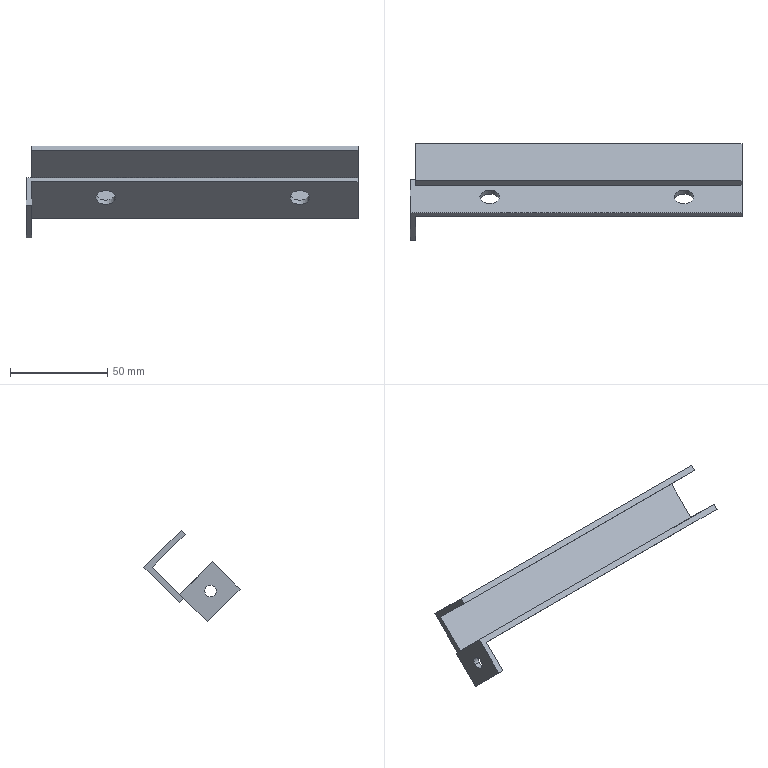Component | SolidWorks | LeftGuardBracket-1 | 1 solid | 20 faces | box 171 x 49.5 x 47.34 mm | volume 38177 mm3 | plane 14 | cylinder 6 | commonest cylinder face diameters 10 x4 6 x2
build123d program:
from build123d import *

# Parameters (mm, degrees)
EXTRUDE_THIN1_DEPTH = 168
SKETCH2_W           = 23.953
SKETCH2_H           = 20
BOSS_EXTRUDE1_DEPTH = 3
SKETCH3_R           = 5
CUT_EXTRUDE1_DEPTH  = 3
SKETCH4_R           = 3
CUT_EXTRUDE2_DEPTH  = 3


with BuildPart() as part:
    # Sketch1 → Extrude-Thin1 (new body)
    with BuildSketch(Plane.XY):
        Polygon((3.367, -34.031), (-23.633, -34.031), (-23.633, -8.031), (3.367, -8.031), (3.367, -11.031), (-20.633, -11.031), (-20.633, -31.031), (3.367, -31.031), align=None)
    extrude(amount=EXTRUDE_THIN1_DEPTH)

    # Sketch2 → Boss-Extrude1 (add)
    with BuildSketch(Plane.XY.offset(168)):
        with Locations((-8.609, -41.031)):
            Rectangle(SKETCH2_W, SKETCH2_H)
    extrude(amount=BOSS_EXTRUDE1_DEPTH)

    # Sketch3 → Cut-Extrude1 (cut)
    with BuildSketch(Plane(origin=(0, -34.031, 0), x_dir=(-1, 0, 0), z_dir=(0, -1, 0))):
        with Locations(Location((8.109, -130, 0), (0, 0, 90))):
            Circle(SKETCH3_R)
        with Locations(Location((8.109, -30, 0), (0, 0, 90))):
            Circle(SKETCH3_R)
    extrude(amount=-CUT_EXTRUDE1_DEPTH, mode=Mode.SUBTRACT)

    # Sketch4 → Cut-Extrude2 (cut)
    with BuildSketch(Plane.XY.offset(171)):
        with Locations((-8.109, -41.031)):
            Circle(SKETCH4_R)
    extrude(amount=-CUT_EXTRUDE2_DEPTH, mode=Mode.SUBTRACT)


solid = part.part

# Placed as in the assembly
solid = solid.moved(Location((-271.55, -172.786, -218.111), (45, -90, 0)))
STEP:
#1=COLOUR_RGB('',0.7922,0.8196,0.9333);
#2=FILL_AREA_STYLE_COLOUR('',#1);
#3=FILL_AREA_STYLE('',(#2));
#4=SURFACE_STYLE_FILL_AREA(#3);
#5=SURFACE_SIDE_STYLE('',(#4));
#6=SURFACE_STYLE_USAGE(.BOTH.,#5);
#7=PRESENTATION_STYLE_ASSIGNMENT((#6));
#8=CARTESIAN_POINT('',(-17.305,-7.636,-10.039));
#9=VERTEX_POINT('',#8);
#10=CARTESIAN_POINT('',(-17.305,-7.803,-9.872));
#11=VERTEX_POINT('',#10);
#12=CARTESIAN_POINT('',(-17.305,-7.719,-9.955));
#13=DIRECTION('',(-1.,0.,0.));
#14=DIRECTION('',(0.,-0.7071,0.7071));
#15=AXIS2_PLACEMENT_3D('',#12,#13,#14);
#16=CIRCLE('',#15,0.1181);
#17=EDGE_CURVE('',#9,#11,#16,.T.);
#18=ORIENTED_EDGE('',*,*,#17,.F.);
#19=CARTESIAN_POINT('',(-17.423,-7.636,-10.039));
#20=VERTEX_POINT('',#19);
#21=CARTESIAN_POINT('',(-17.305,-7.636,-10.039));
#22=DIRECTION('',(-1.,0.,0.));
#23=VECTOR('',#22,39.37);
#24=LINE('',#21,#23);
#25=EDGE_CURVE('',#9,#20,#24,.T.);
#26=ORIENTED_EDGE('',*,*,#25,.T.);
#27=CARTESIAN_POINT('',(-17.423,-7.803,-9.872));
#28=VERTEX_POINT('',#27);
#29=CARTESIAN_POINT('',(-17.423,-7.719,-9.955));
#30=DIRECTION('',(-1.,0.,0.));
#31=DIRECTION('',(0.,-0.7071,0.7071));
#32=AXIS2_PLACEMENT_3D('',#29,#30,#31);
#33=CIRCLE('',#32,0.1181);
#34=EDGE_CURVE('',#20,#28,#33,.T.);
#35=ORIENTED_EDGE('',*,*,#34,.T.);
#36=CARTESIAN_POINT('',(-17.305,-7.803,-9.872));
#37=DIRECTION('',(-1.,0.,0.));
#38=VECTOR('',#37,39.37);
#39=LINE('',#36,#38);
#40=EDGE_CURVE('',#11,#28,#39,.T.);
#41=ORIENTED_EDGE('',*,*,#40,.F.);
#42=EDGE_LOOP('',(#18,#26,#35,#41));
#43=FACE_OUTER_BOUND('',#42,.T.);
#44=CARTESIAN_POINT('',(-17.305,-7.719,-9.955));
#45=DIRECTION('',(-1.,0.,0.));
#46=DIRECTION('',(0.,-0.7071,0.7071));
#47=AXIS2_PLACEMENT_3D('',#44,#45,#46);
#48=CYLINDRICAL_SURFACE('',#47,0.1181);
#49=ADVANCED_FACE('',(#43),#48,.F.);
#50=CARTESIAN_POINT('',(-12.069,-7.441,-9.677));
#51=VERTEX_POINT('',#50);
#52=CARTESIAN_POINT('',(-11.675,-7.441,-9.677));
#53=VERTEX_POINT('',#52);
#54=CARTESIAN_POINT('',(-11.872,-7.441,-9.677));
#55=DIRECTION('',(-0.,-0.7071,-0.7071));
#56=DIRECTION('',(1.,0.,0.));
#57=AXIS2_PLACEMENT_3D('',#54,#55,#56);
#58=CIRCLE('',#57,0.1969);
#59=EDGE_CURVE('',#51,#53,#58,.T.);
#60=ORIENTED_EDGE('',*,*,#59,.F.);
#61=CARTESIAN_POINT('',(-12.069,-7.524,-9.76));
#62=VERTEX_POINT('',#61);
#63=CARTESIAN_POINT('',(-12.069,-7.441,-9.677));
#64=DIRECTION('',(-0.,-0.7071,-0.7071));
#65=VECTOR('',#64,39.37);
#66=LINE('',#63,#65);
#67=EDGE_CURVE('',#51,#62,#66,.T.);
#68=ORIENTED_EDGE('',*,*,#67,.T.);
#69=CARTESIAN_POINT('',(-11.675,-7.524,-9.76));
#70=VERTEX_POINT('',#69);
#71=CARTESIAN_POINT('',(-11.872,-7.524,-9.76));
#72=DIRECTION('',(-0.,-0.7071,-0.7071));
#73=DIRECTION('',(1.,0.,0.));
#74=AXIS2_PLACEMENT_3D('',#71,#72,#73);
#75=CIRCLE('',#74,0.1969);
#76=EDGE_CURVE('',#62,#70,#75,.T.);
#77=ORIENTED_EDGE('',*,*,#76,.T.);
#78=CARTESIAN_POINT('',(-11.675,-7.441,-9.677));
#79=DIRECTION('',(-0.,-0.7071,-0.7071));
#80=VECTOR('',#79,39.37);
#81=LINE('',#78,#80);
#82=EDGE_CURVE('',#53,#70,#81,.T.);
#83=ORIENTED_EDGE('',*,*,#82,.F.);
#84=EDGE_LOOP('',(#60,#68,#77,#83));
#85=FACE_OUTER_BOUND('',#84,.T.);
#86=CARTESIAN_POINT('',(-11.872,-7.441,-9.677));
#87=DIRECTION('',(-0.,-0.7071,-0.7071));
#88=DIRECTION('',(1.,0.,0.));
#89=AXIS2_PLACEMENT_3D('',#86,#87,#88);
#90=CYLINDRICAL_SURFACE('',#89,0.1969);
#91=ADVANCED_FACE('',(#85),#90,.F.);
#92=CARTESIAN_POINT('',(-16.006,-7.441,-9.677));
#93=VERTEX_POINT('',#92);
#94=CARTESIAN_POINT('',(-15.612,-7.441,-9.677));
#95=VERTEX_POINT('',#94);
#96=CARTESIAN_POINT('',(-15.809,-7.441,-9.677));
#97=DIRECTION('',(-0.,-0.7071,-0.7071));
#98=DIRECTION('',(1.,0.,0.));
#99=AXIS2_PLACEMENT_3D('',#96,#97,#98);
#100=CIRCLE('',#99,0.1969);
#101=EDGE_CURVE('',#93,#95,#100,.T.);
#102=ORIENTED_EDGE('',*,*,#101,.F.);
#103=CARTESIAN_POINT('',(-16.006,-7.524,-9.76));
#104=VERTEX_POINT('',#103);
#105=CARTESIAN_POINT('',(-16.006,-7.441,-9.677));
#106=DIRECTION('',(-0.,-0.7071,-0.7071));
#107=VECTOR('',#106,39.37);
#108=LINE('',#105,#107);
#109=EDGE_CURVE('',#93,#104,#108,.T.);
#110=ORIENTED_EDGE('',*,*,#109,.T.);
#111=CARTESIAN_POINT('',(-15.612,-7.524,-9.76));
#112=VERTEX_POINT('',#111);
#113=CARTESIAN_POINT('',(-15.809,-7.524,-9.76));
#114=DIRECTION('',(-0.,-0.7071,-0.7071));
#115=DIRECTION('',(1.,0.,0.));
#116=AXIS2_PLACEMENT_3D('',#113,#114,#115);
#117=CIRCLE('',#116,0.1969);
#118=EDGE_CURVE('',#104,#112,#117,.T.);
#119=ORIENTED_EDGE('',*,*,#118,.T.);
#120=CARTESIAN_POINT('',(-15.612,-7.441,-9.677));
#121=DIRECTION('',(-0.,-0.7071,-0.7071));
#122=VECTOR('',#121,39.37);
#123=LINE('',#120,#122);
#124=EDGE_CURVE('',#95,#112,#123,.T.);
#125=ORIENTED_EDGE('',*,*,#124,.F.);
#126=EDGE_LOOP('',(#102,#110,#119,#125));
#127=FACE_OUTER_BOUND('',#126,.T.);
#128=CARTESIAN_POINT('',(-15.809,-7.441,-9.677));
#129=DIRECTION('',(-0.,-0.7071,-0.7071));
#130=DIRECTION('',(1.,0.,0.));
#131=AXIS2_PLACEMENT_3D('',#128,#129,#130);
#132=CYLINDRICAL_SURFACE('',#131,0.1969);
#133=ADVANCED_FACE('',(#127),#132,.F.);
#134=CARTESIAN_POINT('',(-17.305,-7.093,-10.024));
#135=VERTEX_POINT('',#134);
#136=CARTESIAN_POINT('',(-17.305,-7.177,-10.108));
#137=VERTEX_POINT('',#136);
#138=CARTESIAN_POINT('',(-17.305,-7.093,-10.024));
#139=DIRECTION('',(-0.,-0.7071,-0.7071));
#140=VECTOR('',#139,39.37);
#141=LINE('',#138,#140);
#142=EDGE_CURVE('',#135,#137,#141,.T.);
#143=ORIENTED_EDGE('',*,*,#142,.F.);
#144=CARTESIAN_POINT('',(-17.305,-7.092,-10.025));
#145=VERTEX_POINT('',#144);
#146=CARTESIAN_POINT('',(-17.305,-7.009,-10.109));
#147=DIRECTION('',(0.,0.7071,-0.7071));
#148=VECTOR('',#147,39.37);
#149=LINE('',#146,#148);
#150=EDGE_CURVE('',#135,#145,#149,.T.);
#151=ORIENTED_EDGE('',*,*,#150,.T.);
#152=CARTESIAN_POINT('',(-17.305,-6.535,-9.469));
#153=VERTEX_POINT('',#152);
#154=CARTESIAN_POINT('',(-17.305,-6.452,-9.385));
#155=DIRECTION('',(0.,0.7071,0.7071));
#156=VECTOR('',#155,39.37);
#157=LINE('',#154,#156);
#158=EDGE_CURVE('',#145,#153,#157,.T.);
#159=ORIENTED_EDGE('',*,*,#158,.T.);
#160=CARTESIAN_POINT('',(-17.305,-7.203,-8.8));
#161=VERTEX_POINT('',#160);
#162=CARTESIAN_POINT('',(-17.305,-6.452,-9.552));
#163=DIRECTION('',(-0.,-0.7071,0.7071));
#164=VECTOR('',#163,39.37);
#165=LINE('',#162,#164);
#166=EDGE_CURVE('',#153,#161,#165,.T.);
#167=ORIENTED_EDGE('',*,*,#166,.T.);
#168=CARTESIAN_POINT('',(-17.305,-7.12,-8.717));
#169=VERTEX_POINT('',#168);
#170=CARTESIAN_POINT('',(-17.305,-7.12,-8.717));
#171=DIRECTION('',(-0.,-0.7071,-0.7071));
#172=VECTOR('',#171,39.37);
#173=LINE('',#170,#172);
#174=EDGE_CURVE('',#169,#161,#173,.T.);
#175=ORIENTED_EDGE('',*,*,#174,.F.);
#176=CARTESIAN_POINT('',(-17.305,-6.368,-9.469));
#177=VERTEX_POINT('',#176);
#178=CARTESIAN_POINT('',(-17.305,-6.368,-9.469));
#179=DIRECTION('',(-0.,-0.7071,0.7071));
#180=VECTOR('',#179,39.37);
#181=LINE('',#178,#180);
#182=EDGE_CURVE('',#177,#169,#181,.T.);
#183=ORIENTED_EDGE('',*,*,#182,.F.);
#184=CARTESIAN_POINT('',(-17.305,-7.092,-10.192));
#185=VERTEX_POINT('',#184);
#186=CARTESIAN_POINT('',(-17.305,-6.368,-9.469));
#187=DIRECTION('',(0.,0.7071,0.7071));
#188=VECTOR('',#187,39.37);
#189=LINE('',#186,#188);
#190=EDGE_CURVE('',#185,#177,#189,.T.);
#191=ORIENTED_EDGE('',*,*,#190,.F.);
#192=CARTESIAN_POINT('',(-17.305,-7.092,-10.192));
#193=DIRECTION('',(0.,0.7071,-0.7071));
#194=VECTOR('',#193,39.37);
#195=LINE('',#192,#194);
#196=EDGE_CURVE('',#137,#185,#195,.T.);
#197=ORIENTED_EDGE('',*,*,#196,.F.);
#198=EDGE_LOOP('',(#143,#151,#159,#167,#175,#183,#191,#197));
#199=FACE_OUTER_BOUND('',#198,.T.);
#200=CARTESIAN_POINT('',(-17.305,-6.803,-8.587));
#201=DIRECTION('',(1.,-0.,-0.));
#202=DIRECTION('',(0.,0.7071,-0.7071));
#203=AXIS2_PLACEMENT_3D('',#200,#201,#202);
#204=PLANE('',#203);
#205=ADVANCED_FACE('',(#199),#204,.F.);
#206=CARTESIAN_POINT('',(-10.691,-6.535,-9.469));
#207=VERTEX_POINT('',#206);
#208=CARTESIAN_POINT('',(-10.691,-7.203,-8.8));
#209=VERTEX_POINT('',#208);
#210=CARTESIAN_POINT('',(-10.691,-6.452,-9.552));
#211=DIRECTION('',(-0.,-0.7071,0.7071));
#212=VECTOR('',#211,39.37);
#213=LINE('',#210,#212);
#214=EDGE_CURVE('',#207,#209,#213,.T.);
#215=ORIENTED_EDGE('',*,*,#214,.T.);
#216=CARTESIAN_POINT('',(-17.305,-7.203,-8.8));
#217=DIRECTION('',(1.,-0.,0.));
#218=VECTOR('',#217,39.37);
#219=LINE('',#216,#218);
#220=EDGE_CURVE('',#161,#209,#219,.T.);
#221=ORIENTED_EDGE('',*,*,#220,.F.);
#222=ORIENTED_EDGE('',*,*,#166,.F.);
#223=CARTESIAN_POINT('',(-17.305,-6.535,-9.469));
#224=DIRECTION('',(1.,-0.,0.));
#225=VECTOR('',#224,39.37);
#226=LINE('',#223,#225);
#227=EDGE_CURVE('',#153,#207,#226,.T.);
#228=ORIENTED_EDGE('',*,*,#227,.T.);
#229=EDGE_LOOP('',(#215,#221,#222,#228));
#230=FACE_OUTER_BOUND('',#229,.T.);
#231=CARTESIAN_POINT('',(-17.305,-6.452,-9.552));
#232=DIRECTION('',(0.,0.7071,0.7071));
#233=DIRECTION('',(0.,0.7071,-0.7071));
#234=AXIS2_PLACEMENT_3D('',#231,#232,#233);
#235=PLANE('',#234);
#236=ADVANCED_FACE('',(#230),#235,.F.);
#237=CARTESIAN_POINT('',(-10.691,-7.12,-8.717));
#238=VERTEX_POINT('',#237);
#239=CARTESIAN_POINT('',(-10.691,-7.12,-8.717));
#240=DIRECTION('',(-0.,-0.7071,-0.7071));
#241=VECTOR('',#240,39.37);
#242=LINE('',#239,#241);
#243=EDGE_CURVE('',#238,#209,#242,.T.);
#244=ORIENTED_EDGE('',*,*,#243,.F.);
#245=CARTESIAN_POINT('',(-17.305,-7.12,-8.717));
#246=DIRECTION('',(1.,-0.,0.));
#247=VECTOR('',#246,39.37);
#248=LINE('',#245,#247);
#249=EDGE_CURVE('',#169,#238,#248,.T.);
#250=ORIENTED_EDGE('',*,*,#249,.F.);
#251=ORIENTED_EDGE('',*,*,#174,.T.);
#252=ORIENTED_EDGE('',*,*,#220,.T.);
#253=EDGE_LOOP('',(#244,#250,#251,#252));
#254=FACE_OUTER_BOUND('',#253,.T.);
#255=CARTESIAN_POINT('',(-17.305,-7.12,-8.717));
#256=DIRECTION('',(-0.,-0.7071,0.7071));
#257=DIRECTION('',(1.,-0.,0.));
#258=AXIS2_PLACEMENT_3D('',#255,#256,#257);
#259=PLANE('',#258);
#260=ADVANCED_FACE('',(#254),#259,.T.);
#261=CARTESIAN_POINT('',(-10.691,-6.368,-9.469));
#262=VERTEX_POINT('',#261);
#263=CARTESIAN_POINT('',(-10.691,-6.368,-9.469));
#264=DIRECTION('',(-0.,-0.7071,0.7071));
#265=VECTOR('',#264,39.37);
#266=LINE('',#263,#265);
#267=EDGE_CURVE('',#262,#238,#266,.T.);
#268=ORIENTED_EDGE('',*,*,#267,.F.);
#269=CARTESIAN_POINT('',(-17.305,-6.368,-9.469));
#270=DIRECTION('',(1.,-0.,0.));
#271=VECTOR('',#270,39.37);
#272=LINE('',#269,#271);
#273=EDGE_CURVE('',#177,#262,#272,.T.);
#274=ORIENTED_EDGE('',*,*,#273,.F.);
#275=ORIENTED_EDGE('',*,*,#182,.T.);
#276=ORIENTED_EDGE('',*,*,#249,.T.);
#277=EDGE_LOOP('',(#268,#274,#275,#276));
#278=FACE_OUTER_BOUND('',#277,.T.);
#279=CARTESIAN_POINT('',(-17.305,-6.368,-9.469));
#280=DIRECTION('',(0.,0.7071,0.7071));
#281=DIRECTION('',(0.,0.7071,-0.7071));
#282=AXIS2_PLACEMENT_3D('',#279,#280,#281);
#283=PLANE('',#282);
#284=ADVANCED_FACE('',(#278),#283,.T.);
#285=CARTESIAN_POINT('',(-10.691,-7.092,-10.192));
#286=VERTEX_POINT('',#285);
#287=CARTESIAN_POINT('',(-10.691,-6.368,-9.469));
#288=DIRECTION('',(0.,0.7071,0.7071));
#289=VECTOR('',#288,39.37);
#290=LINE('',#287,#289);
#291=EDGE_CURVE('',#286,#262,#290,.T.);
#292=ORIENTED_EDGE('',*,*,#291,.F.);
#293=CARTESIAN_POINT('',(-17.305,-7.092,-10.192));
#294=DIRECTION('',(1.,-0.,0.));
#295=VECTOR('',#294,39.37);
#296=LINE('',#293,#295);
#297=EDGE_CURVE('',#185,#286,#296,.T.);
#298=ORIENTED_EDGE('',*,*,#297,.F.);
#299=ORIENTED_EDGE('',*,*,#190,.T.);
#300=ORIENTED_EDGE('',*,*,#273,.T.);
#301=EDGE_LOOP('',(#292,#298,#299,#300));
#302=FACE_OUTER_BOUND('',#301,.T.);
#303=CARTESIAN_POINT('',(-17.305,-6.368,-9.469));
#304=DIRECTION('',(0.,0.7071,-0.7071));
#305=DIRECTION('',(-0.,-0.7071,-0.7071));
#306=AXIS2_PLACEMENT_3D('',#303,#304,#305);
#307=PLANE('',#306);
#308=ADVANCED_FACE('',(#302),#307,.T.);
#309=CARTESIAN_POINT('',(-11.872,-7.524,-9.76));
#310=DIRECTION('',(-0.,-0.7071,-0.7071));
#311=DIRECTION('',(1.,0.,0.));
#312=AXIS2_PLACEMENT_3D('',#309,#310,#311);
#313=CIRCLE('',#312,0.1969);
#314=EDGE_CURVE('',#70,#62,#313,.T.);
#315=ORIENTED_EDGE('',*,*,#314,.F.);
#316=ORIENTED_EDGE('',*,*,#76,.F.);
#317=EDGE_LOOP('',(#315,#316));
#318=FACE_BOUND('',#317,.T.);
#319=CARTESIAN_POINT('',(-15.809,-7.524,-9.76));
#320=DIRECTION('',(-0.,-0.7071,-0.7071));
#321=DIRECTION('',(1.,0.,0.));
#322=AXIS2_PLACEMENT_3D('',#319,#320,#321);
#323=CIRCLE('',#322,0.1969);
#324=EDGE_CURVE('',#112,#104,#323,.T.);
#325=ORIENTED_EDGE('',*,*,#324,.F.);
#326=ORIENTED_EDGE('',*,*,#118,.F.);
#327=EDGE_LOOP('',(#325,#326));
#328=FACE_BOUND('',#327,.T.);
#329=CARTESIAN_POINT('',(-10.691,-7.844,-9.441));
#330=VERTEX_POINT('',#329);
#331=CARTESIAN_POINT('',(-10.691,-7.092,-10.192));
#332=DIRECTION('',(0.,0.7071,-0.7071));
#333=VECTOR('',#332,39.37);
#334=LINE('',#331,#333);
#335=EDGE_CURVE('',#330,#286,#334,.T.);
#336=ORIENTED_EDGE('',*,*,#335,.F.);
#337=CARTESIAN_POINT('',(-17.305,-7.844,-9.441));
#338=VERTEX_POINT('',#337);
#339=CARTESIAN_POINT('',(-17.305,-7.844,-9.441));
#340=DIRECTION('',(1.,-0.,0.));
#341=VECTOR('',#340,39.37);
#342=LINE('',#339,#341);
#343=EDGE_CURVE('',#338,#330,#342,.T.);
#344=ORIENTED_EDGE('',*,*,#343,.F.);
#345=CARTESIAN_POINT('',(-17.305,-7.092,-10.192));
#346=DIRECTION('',(0.,0.7071,-0.7071));
#347=VECTOR('',#346,39.37);
#348=LINE('',#345,#347);
#349=EDGE_CURVE('',#338,#137,#348,.T.);
#350=ORIENTED_EDGE('',*,*,#349,.T.);
#351=ORIENTED_EDGE('',*,*,#196,.T.);
#352=ORIENTED_EDGE('',*,*,#297,.T.);
#353=EDGE_LOOP('',(#336,#344,#350,#351,#352));
#354=FACE_OUTER_BOUND('',#353,.T.);
#355=CARTESIAN_POINT('',(-17.305,-7.092,-10.192));
#356=DIRECTION('',(-0.,-0.7071,-0.7071));
#357=DIRECTION('',(1.,-0.,0.));
#358=AXIS2_PLACEMENT_3D('',#355,#356,#357);
#359=PLANE('',#358);
#360=ADVANCED_FACE('',(#318,#328,#354),#359,.T.);
#361=CARTESIAN_POINT('',(-10.691,-7.76,-9.357));
#362=VERTEX_POINT('',#361);
#363=CARTESIAN_POINT('',(-10.691,-7.76,-9.357));
#364=DIRECTION('',(-0.,-0.7071,-0.7071));
#365=VECTOR('',#364,39.37);
#366=LINE('',#363,#365);
#367=EDGE_CURVE('',#362,#330,#366,.T.);
#368=ORIENTED_EDGE('',*,*,#367,.F.);
#369=CARTESIAN_POINT('',(-17.423,-7.76,-9.357));
#370=VERTEX_POINT('',#369);
#371=CARTESIAN_POINT('',(-17.305,-7.76,-9.357));
#372=DIRECTION('',(1.,-0.,0.));
#373=VECTOR('',#372,39.37);
#374=LINE('',#371,#373);
#375=EDGE_CURVE('',#370,#362,#374,.T.);
#376=ORIENTED_EDGE('',*,*,#375,.F.);
#377=CARTESIAN_POINT('',(-17.423,-8.317,-9.914));
#378=VERTEX_POINT('',#377);
#379=CARTESIAN_POINT('',(-17.423,-7.76,-9.357));
#380=DIRECTION('',(0.,0.7071,0.7071));
#381=VECTOR('',#380,39.37);
#382=LINE('',#379,#381);
#383=EDGE_CURVE('',#378,#370,#382,.T.);
#384=ORIENTED_EDGE('',*,*,#383,.F.);
#385=CARTESIAN_POINT('',(-17.305,-8.317,-9.914));
#386=VERTEX_POINT('',#385);
#387=CARTESIAN_POINT('',(-17.423,-8.317,-9.914));
#388=DIRECTION('',(1.,-0.,0.));
#389=VECTOR('',#388,39.37);
#390=LINE('',#387,#389);
#391=EDGE_CURVE('',#378,#386,#390,.T.);
#392=ORIENTED_EDGE('',*,*,#391,.T.);
#393=CARTESIAN_POINT('',(-17.305,-7.76,-9.357));
#394=DIRECTION('',(0.,0.7071,0.7071));
#395=VECTOR('',#394,39.37);
#396=LINE('',#393,#395);
#397=EDGE_CURVE('',#386,#338,#396,.T.);
#398=ORIENTED_EDGE('',*,*,#397,.T.);
#399=ORIENTED_EDGE('',*,*,#343,.T.);
#400=EDGE_LOOP('',(#368,#376,#384,#392,#398,#399));
#401=FACE_OUTER_BOUND('',#400,.T.);
#402=CARTESIAN_POINT('',(-17.305,-7.76,-9.357));
#403=DIRECTION('',(-0.,-0.7071,0.7071));
#404=DIRECTION('',(1.,-0.,0.));
#405=AXIS2_PLACEMENT_3D('',#402,#403,#404);
#406=PLANE('',#405);
#407=ADVANCED_FACE('',(#401),#406,.T.);
#408=CARTESIAN_POINT('',(-11.872,-7.441,-9.677));
#409=DIRECTION('',(-0.,-0.7071,-0.7071));
#410=DIRECTION('',(1.,0.,0.));
#411=AXIS2_PLACEMENT_3D('',#408,#409,#410);
#412=CIRCLE('',#411,0.1969);
#413=EDGE_CURVE('',#53,#51,#412,.T.);
#414=ORIENTED_EDGE('',*,*,#413,.T.);
#415=ORIENTED_EDGE('',*,*,#59,.T.);
#416=EDGE_LOOP('',(#414,#415));
#417=FACE_BOUND('',#416,.T.);
#418=CARTESIAN_POINT('',(-15.809,-7.441,-9.677));
#419=DIRECTION('',(-0.,-0.7071,-0.7071));
#420=DIRECTION('',(1.,0.,0.));
#421=AXIS2_PLACEMENT_3D('',#418,#419,#420);
#422=CIRCLE('',#421,0.1969);
#423=EDGE_CURVE('',#95,#93,#422,.T.);
#424=ORIENTED_EDGE('',*,*,#423,.T.);
#425=ORIENTED_EDGE('',*,*,#101,.T.);
#426=EDGE_LOOP('',(#424,#425));
#427=FACE_BOUND('',#426,.T.);
#428=CARTESIAN_POINT('',(-10.691,-7.092,-10.025));
#429=VERTEX_POINT('',#428);
#430=CARTESIAN_POINT('',(-10.691,-7.009,-10.109));
#431=DIRECTION('',(0.,0.7071,-0.7071));
#432=VECTOR('',#431,39.37);
#433=LINE('',#430,#432);
#434=EDGE_CURVE('',#362,#429,#433,.T.);
#435=ORIENTED_EDGE('',*,*,#434,.T.);
#436=CARTESIAN_POINT('',(-17.305,-7.092,-10.025));
#437=DIRECTION('',(1.,-0.,0.));
#438=VECTOR('',#437,39.37);
#439=LINE('',#436,#438);
#440=EDGE_CURVE('',#145,#429,#439,.T.);
#441=ORIENTED_EDGE('',*,*,#440,.F.);
#442=ORIENTED_EDGE('',*,*,#150,.F.);
#443=CARTESIAN_POINT('',(-17.423,-7.093,-10.024));
#444=VERTEX_POINT('',#443);
#445=CARTESIAN_POINT('',(-17.423,-7.093,-10.024));
#446=DIRECTION('',(1.,-0.,0.));
#447=VECTOR('',#446,39.37);
#448=LINE('',#445,#447);
#449=EDGE_CURVE('',#444,#135,#448,.T.);
#450=ORIENTED_EDGE('',*,*,#449,.F.);
#451=CARTESIAN_POINT('',(-17.423,-7.76,-9.357));
#452=DIRECTION('',(0.,0.7071,-0.7071));
#453=VECTOR('',#452,39.37);
#454=LINE('',#451,#453);
#455=EDGE_CURVE('',#370,#444,#454,.T.);
#456=ORIENTED_EDGE('',*,*,#455,.F.);
#457=ORIENTED_EDGE('',*,*,#375,.T.);
#458=EDGE_LOOP('',(#435,#441,#442,#450,#456,#457));
#459=FACE_OUTER_BOUND('',#458,.T.);
#460=CARTESIAN_POINT('',(-17.305,-7.009,-10.109));
#461=DIRECTION('',(-0.,-0.7071,-0.7071));
#462=DIRECTION('',(1.,-0.,0.));
#463=AXIS2_PLACEMENT_3D('',#460,#461,#462);
#464=PLANE('',#463);
#465=ADVANCED_FACE('',(#417,#427,#459),#464,.F.);
#466=CARTESIAN_POINT('',(-10.691,-6.452,-9.385));
#467=DIRECTION('',(0.,0.7071,0.7071));
#468=VECTOR('',#467,39.37);
#469=LINE('',#466,#468);
#470=EDGE_CURVE('',#429,#207,#469,.T.);
#471=ORIENTED_EDGE('',*,*,#470,.T.);
#472=ORIENTED_EDGE('',*,*,#227,.F.);
#473=ORIENTED_EDGE('',*,*,#158,.F.);
#474=ORIENTED_EDGE('',*,*,#440,.T.);
#475=EDGE_LOOP('',(#471,#472,#473,#474));
#476=FACE_OUTER_BOUND('',#475,.T.);
#477=CARTESIAN_POINT('',(-17.305,-6.452,-9.385));
#478=DIRECTION('',(0.,0.7071,-0.7071));
#479=DIRECTION('',(-0.,-0.7071,-0.7071));
#480=AXIS2_PLACEMENT_3D('',#477,#478,#479);
#481=PLANE('',#480);
#482=ADVANCED_FACE('',(#476),#481,.F.);
#483=ORIENTED_EDGE('',*,*,#214,.F.);
#484=ORIENTED_EDGE('',*,*,#470,.F.);
#485=ORIENTED_EDGE('',*,*,#434,.F.);
#486=ORIENTED_EDGE('',*,*,#367,.T.);
#487=ORIENTED_EDGE('',*,*,#335,.T.);
#488=ORIENTED_EDGE('',*,*,#291,.T.);
#489=ORIENTED_EDGE('',*,*,#267,.T.);
#490=ORIENTED_EDGE('',*,*,#243,.T.);
#491=EDGE_LOOP('',(#483,#484,#485,#486,#487,#488,#489,#490));
#492=FACE_OUTER_BOUND('',#491,.T.);
#493=CARTESIAN_POINT('',(-10.691,-6.803,-8.587));
#494=DIRECTION('',(1.,-0.,-0.));
#495=DIRECTION('',(0.,0.7071,-0.7071));
#496=AXIS2_PLACEMENT_3D('',#493,#494,#495);
#497=PLANE('',#496);
#498=ADVANCED_FACE('',(#492),#497,.T.);
#499=CARTESIAN_POINT('',(-17.305,-7.719,-9.955));
#500=DIRECTION('',(-1.,0.,0.));
#501=DIRECTION('',(0.,-0.7071,0.7071));
#502=AXIS2_PLACEMENT_3D('',#499,#500,#501);
#503=CIRCLE('',#502,0.1181);
#504=EDGE_CURVE('',#11,#9,#503,.T.);
#505=ORIENTED_EDGE('',*,*,#504,.T.);
#506=ORIENTED_EDGE('',*,*,#17,.T.);
#507=EDGE_LOOP('',(#505,#506));
#508=FACE_BOUND('',#507,.T.);
#509=ORIENTED_EDGE('',*,*,#349,.F.);
#510=ORIENTED_EDGE('',*,*,#397,.F.);
#511=CARTESIAN_POINT('',(-17.305,-7.65,-10.581));
#512=VERTEX_POINT('',#511);
#513=CARTESIAN_POINT('',(-17.305,-8.317,-9.914));
#514=DIRECTION('',(-0.,-0.7071,0.7071));
#515=VECTOR('',#514,39.37);
#516=LINE('',#513,#515);
#517=EDGE_CURVE('',#512,#386,#516,.T.);
#518=ORIENTED_EDGE('',*,*,#517,.F.);
#519=CARTESIAN_POINT('',(-17.305,-7.093,-10.024));
#520=DIRECTION('',(-0.,-0.7071,-0.7071));
#521=VECTOR('',#520,39.37);
#522=LINE('',#519,#521);
#523=EDGE_CURVE('',#137,#512,#522,.T.);
#524=ORIENTED_EDGE('',*,*,#523,.F.);
#525=EDGE_LOOP('',(#509,#510,#518,#524));
#526=FACE_OUTER_BOUND('',#525,.T.);
#527=CARTESIAN_POINT('',(-17.305,-6.803,-8.587));
#528=DIRECTION('',(1.,-0.,-0.));
#529=DIRECTION('',(0.,0.7071,-0.7071));
#530=AXIS2_PLACEMENT_3D('',#527,#528,#529);
#531=PLANE('',#530);
#532=ADVANCED_FACE('',(#508,#526),#531,.T.);
#533=ORIENTED_EDGE('',*,*,#142,.T.);
#534=ORIENTED_EDGE('',*,*,#523,.T.);
#535=CARTESIAN_POINT('',(-17.423,-7.65,-10.581));
#536=VERTEX_POINT('',#535);
#537=CARTESIAN_POINT('',(-17.423,-7.65,-10.581));
#538=DIRECTION('',(1.,-0.,0.));
#539=VECTOR('',#538,39.37);
#540=LINE('',#537,#539);
#541=EDGE_CURVE('',#536,#512,#540,.T.);
#542=ORIENTED_EDGE('',*,*,#541,.F.);
#543=CARTESIAN_POINT('',(-17.423,-7.093,-10.024));
#544=DIRECTION('',(-0.,-0.7071,-0.7071));
#545=VECTOR('',#544,39.37);
#546=LINE('',#543,#545);
#547=EDGE_CURVE('',#444,#536,#546,.T.);
#548=ORIENTED_EDGE('',*,*,#547,.F.);
#549=ORIENTED_EDGE('',*,*,#449,.T.);
#550=EDGE_LOOP('',(#533,#534,#542,#548,#549));
#551=FACE_OUTER_BOUND('',#550,.T.);
#552=CARTESIAN_POINT('',(-17.423,-7.093,-10.024));
#553=DIRECTION('',(-0.,-0.7071,0.7071));
#554=DIRECTION('',(0.,0.7071,0.7071));
#555=AXIS2_PLACEMENT_3D('',#552,#553,#554);
#556=PLANE('',#555);
#557=ADVANCED_FACE('',(#551),#556,.F.);
#558=ORIENTED_EDGE('',*,*,#517,.T.);
#559=ORIENTED_EDGE('',*,*,#391,.F.);
#560=CARTESIAN_POINT('',(-17.423,-8.317,-9.914));
#561=DIRECTION('',(-0.,-0.7071,0.7071));
#562=VECTOR('',#561,39.37);
#563=LINE('',#560,#562);
#564=EDGE_CURVE('',#536,#378,#563,.T.);
#565=ORIENTED_EDGE('',*,*,#564,.F.);
#566=ORIENTED_EDGE('',*,*,#541,.T.);
#567=EDGE_LOOP('',(#558,#559,#565,#566));
#568=FACE_OUTER_BOUND('',#567,.T.);
#569=CARTESIAN_POINT('',(-17.423,-8.317,-9.914));
#570=DIRECTION('',(0.,0.7071,0.7071));
#571=DIRECTION('',(-1.,0.,0.));
#572=AXIS2_PLACEMENT_3D('',#569,#570,#571);
#573=PLANE('',#572);
#574=ADVANCED_FACE('',(#568),#573,.F.);
#575=CARTESIAN_POINT('',(-17.423,-7.719,-9.955));
#576=DIRECTION('',(-1.,0.,0.));
#577=DIRECTION('',(0.,-0.7071,0.7071));
#578=AXIS2_PLACEMENT_3D('',#575,#576,#577);
#579=CIRCLE('',#578,0.1181);
#580=EDGE_CURVE('',#28,#20,#579,.T.);
#581=ORIENTED_EDGE('',*,*,#580,.F.);
#582=ORIENTED_EDGE('',*,*,#34,.F.);
#583=EDGE_LOOP('',(#581,#582));
#584=FACE_BOUND('',#583,.T.);
#585=ORIENTED_EDGE('',*,*,#383,.T.);
#586=ORIENTED_EDGE('',*,*,#455,.T.);
#587=ORIENTED_EDGE('',*,*,#547,.T.);
#588=ORIENTED_EDGE('',*,*,#564,.T.);
#589=EDGE_LOOP('',(#585,#586,#587,#588));
#590=FACE_OUTER_BOUND('',#589,.T.);
#591=CARTESIAN_POINT('',(-17.423,-6.803,-8.587));
#592=DIRECTION('',(1.,-0.,-0.));
#593=DIRECTION('',(0.,0.7071,-0.7071));
#594=AXIS2_PLACEMENT_3D('',#591,#592,#593);
#595=PLANE('',#594);
#596=ADVANCED_FACE('',(#584,#590),#595,.F.);
#597=ORIENTED_EDGE('',*,*,#109,.F.);
#598=ORIENTED_EDGE('',*,*,#423,.F.);
#599=ORIENTED_EDGE('',*,*,#124,.T.);
#600=ORIENTED_EDGE('',*,*,#324,.T.);
#601=EDGE_LOOP('',(#597,#598,#599,#600));
#602=FACE_OUTER_BOUND('',#601,.T.);
#603=CARTESIAN_POINT('',(-15.809,-7.441,-9.677));
#604=DIRECTION('',(-0.,-0.7071,-0.7071));
#605=DIRECTION('',(1.,0.,0.));
#606=AXIS2_PLACEMENT_3D('',#603,#604,#605);
#607=CYLINDRICAL_SURFACE('',#606,0.1969);
#608=ADVANCED_FACE('',(#602),#607,.F.);
#609=ORIENTED_EDGE('',*,*,#67,.F.);
#610=ORIENTED_EDGE('',*,*,#413,.F.);
#611=ORIENTED_EDGE('',*,*,#82,.T.);
#612=ORIENTED_EDGE('',*,*,#314,.T.);
#613=EDGE_LOOP('',(#609,#610,#611,#612));
#614=FACE_OUTER_BOUND('',#613,.T.);
#615=CARTESIAN_POINT('',(-11.872,-7.441,-9.677));
#616=DIRECTION('',(-0.,-0.7071,-0.7071));
#617=DIRECTION('',(1.,0.,0.));
#618=AXIS2_PLACEMENT_3D('',#615,#616,#617);
#619=CYLINDRICAL_SURFACE('',#618,0.1969);
#620=ADVANCED_FACE('',(#614),#619,.F.);
#621=ORIENTED_EDGE('',*,*,#25,.F.);
#622=ORIENTED_EDGE('',*,*,#504,.F.);
#623=ORIENTED_EDGE('',*,*,#40,.T.);
#624=ORIENTED_EDGE('',*,*,#580,.T.);
#625=EDGE_LOOP('',(#621,#622,#623,#624));
#626=FACE_OUTER_BOUND('',#625,.T.);
#627=CARTESIAN_POINT('',(-17.305,-7.719,-9.955));
#628=DIRECTION('',(-1.,0.,0.));
#629=DIRECTION('',(0.,-0.7071,0.7071));
#630=AXIS2_PLACEMENT_3D('',#627,#628,#629);
#631=CYLINDRICAL_SURFACE('',#630,0.1181);
#632=ADVANCED_FACE('',(#626),#631,.F.);
#633=CLOSED_SHELL('',(#49,#91,#133,#205,#236,#260,#284,#308,#360,#407,#465,#482,#498,#532,#557,#574,#596,#608,#620,#632));
#634=MANIFOLD_SOLID_BREP('',#633);
#635=STYLED_ITEM('',(#7),#634);
#636=(LENGTH_UNIT()NAMED_UNIT(*)SI_UNIT($,.METRE.));
#637=LENGTH_MEASURE_WITH_UNIT(LENGTH_MEASURE(0.0254),#636);
#638=DIMENSIONAL_EXPONENTS(1.,0.,0.,0.,0.,0.,0.);
#639=(CONVERSION_BASED_UNIT('',#637)LENGTH_UNIT()NAMED_UNIT(#638));
#640=UNCERTAINTY_MEASURE_WITH_UNIT(LENGTH_MEASURE(0.00001),#639,'','');
#641=(NAMED_UNIT(*)PLANE_ANGLE_UNIT()SI_UNIT($,.RADIAN.));
#642=(NAMED_UNIT(*)SI_UNIT($,.STERADIAN.)SOLID_ANGLE_UNIT());
#643=(GEOMETRIC_REPRESENTATION_CONTEXT(3)GLOBAL_UNCERTAINTY_ASSIGNED_CONTEXT((#640))GLOBAL_UNIT_ASSIGNED_CONTEXT((#639,#641,#642))REPRESENTATION_CONTEXT('',''));
#644=MECHANICAL_DESIGN_GEOMETRIC_PRESENTATION_REPRESENTATION('',(#635),#643);
#645=CARTESIAN_POINT('',(0.,0.,0.));
#646=DIRECTION('',(0.,0.,1.));
#647=DIRECTION('',(1.,0.,0.));
#648=AXIS2_PLACEMENT_3D('',#645,#646,#647);
#649=(LENGTH_UNIT()NAMED_UNIT(*)SI_UNIT($,.METRE.));
#650=LENGTH_MEASURE_WITH_UNIT(LENGTH_MEASURE(0.0254),#649);
#651=DIMENSIONAL_EXPONENTS(1.,0.,0.,0.,0.,0.,0.);
#652=(CONVERSION_BASED_UNIT('',#650)LENGTH_UNIT()NAMED_UNIT(#651));
#653=UNCERTAINTY_MEASURE_WITH_UNIT(LENGTH_MEASURE(0.00001),#652,'','');
#654=(NAMED_UNIT(*)PLANE_ANGLE_UNIT()SI_UNIT($,.RADIAN.));
#655=(NAMED_UNIT(*)SI_UNIT($,.STERADIAN.)SOLID_ANGLE_UNIT());
#656=(GEOMETRIC_REPRESENTATION_CONTEXT(3)GLOBAL_UNCERTAINTY_ASSIGNED_CONTEXT((#653))GLOBAL_UNIT_ASSIGNED_CONTEXT((#652,#654,#655))REPRESENTATION_CONTEXT('',''));
#657=ADVANCED_BREP_SHAPE_REPRESENTATION('',(#634,#648),#656);
#658=PRESENTATION_LAYER_ASSIGNMENT('','',(#635));